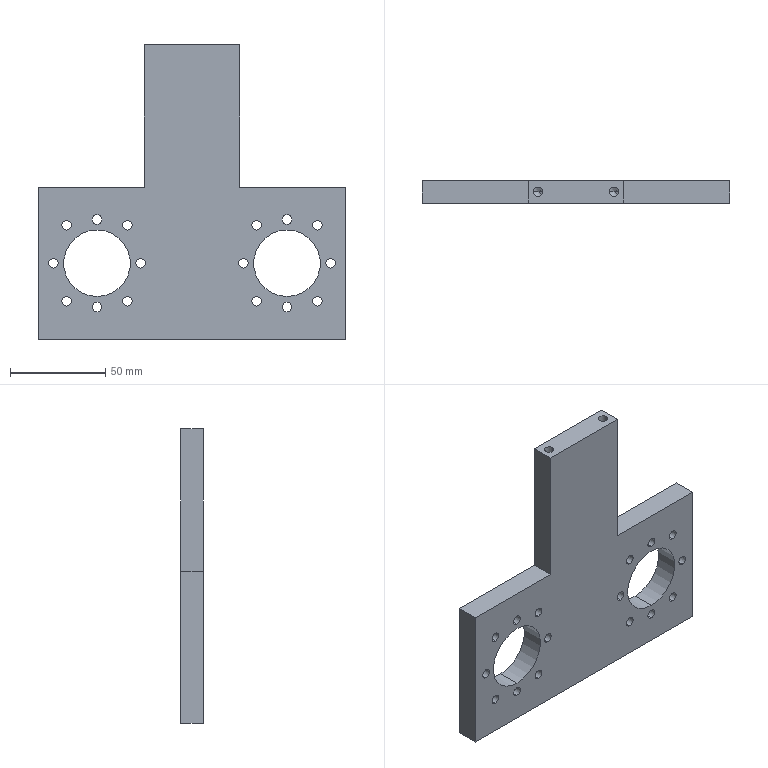Component | SolidWorks | CouplingPlate-1 | 1 solid | 54 faces | box 162 x 12 x 155 mm | volume 173051 mm3 | cylinder 40 | plane 10 | cone 4 | commonest cylinder face diameters 5 x36 35 x4
build123d program:
from build123d import *

# Parameters (mm, degrees)
SKETCH1_R                  = 17.5
EXTRUDE1_DEPTH             = 12
M6_TAPPED_HOLE1_D          = 5
M6_TAPPED_HOLE1_DEPTH      = 15
M6_TAPPED_HOLE1_TIP        = 1.502
M6_TAPPED_HOLE2_AT_2_COUNT = 2
M6_TAPPED_HOLE2_AT_2_PITCH = 32
M6_TAPPED_HOLE2_AT_3_COUNT = 2
M6_TAPPED_HOLE2_AT_3_PITCH = 51.225
M6_TAPPED_HOLE2_AT_4_COUNT = 2
M6_TAPPED_HOLE2_AT_4_PITCH = 40
M6_TAPPED_HOLE2_AT_5_COUNT = 2
M6_TAPPED_HOLE2_AT_5_PITCH = 45.88
M6_TAPPED_HOLE2_AT_6_COUNT = 2
M6_TAPPED_HOLE2_AT_6_PITCH = 43.829
M6_TAPPED_HOLE2_AT_7_COUNT = 2
M6_TAPPED_HOLE2_AT_7_PITCH = 16.279
M6_TAPPED_HOLE2_AT_8_COUNT = 2
M6_TAPPED_HOLE2_AT_8_PITCH = 21.19


with BuildPart() as part:
    # Sketch1 → Extrude1 (new body)
    with BuildSketch(Plane(origin=(0, 0, 0), x_dir=(1, 0, 0), z_dir=(0, 1, 0))):
        Polygon((-81, 80), (81, 80), (81, 0), (25, 0), (25, -75), (-25, -75), (-25, 0), (-81, 0), align=None)
        with Locations(Location((50, 40, 0), (0, 0, 270))):
            Circle(SKETCH1_R, mode=Mode.SUBTRACT)
        with Locations(Location((-50, 40, 0), (0, 0, 90))):
            Circle(SKETCH1_R, mode=Mode.SUBTRACT)
    extrude(amount=EXTRUDE1_DEPTH)

    # M6 Tapped Hole1
    with Locations(Plane.XY.offset(75)):
        with Locations((-20, 6), (20, 6)):
            Hole(M6_TAPPED_HOLE1_D / 2, depth=M6_TAPPED_HOLE1_DEPTH)
            with Locations((0, 0, -(M6_TAPPED_HOLE1_DEPTH + M6_TAPPED_HOLE1_TIP / 2))):  # 118° drill point
                Cone(0, M6_TAPPED_HOLE1_D / 2, M6_TAPPED_HOLE1_TIP, mode=Mode.SUBTRACT)

    # Sketch4 → M6 Tapped Hole2 (revolve, cut)
    with BuildSketch(Plane(origin=(-66, 12, -60), x_dir=(0, 0, 1), z_dir=(1, 0, 0))):
        Polygon((0, 0), (0, 16.502), (2.5, 15), (2.5, 0), align=None)
    m6_tapped_hole2 = revolve(axis=Axis((-66, 18.35, -60), (0, -1, 0)), mode=Mode.SUBTRACT)

    # M6 Tapped Hole2 at 2: M6 Tapped Hole2 ×2
    with Locations(*[(i * M6_TAPPED_HOLE2_AT_2_PITCH, 0, 0) for i in range(1, M6_TAPPED_HOLE2_AT_2_COUNT)]):
        add(m6_tapped_hole2, mode=Mode.SUBTRACT)

    # M6 Tapped Hole2 at 3: M6 Tapped Hole2 ×2
    with Locations(*[Vector(0.6247, 0, 0.7809) * (i * M6_TAPPED_HOLE2_AT_3_PITCH) for i in range(1, M6_TAPPED_HOLE2_AT_3_COUNT)]):
        add(m6_tapped_hole2, mode=Mode.SUBTRACT)

    # M6 Tapped Hole2 at 4: M6 Tapped Hole2 ×2
    with Locations(*[(0, 0, i * M6_TAPPED_HOLE2_AT_4_PITCH) for i in range(1, M6_TAPPED_HOLE2_AT_4_COUNT)]):
        add(m6_tapped_hole2, mode=Mode.SUBTRACT)

    # M6 Tapped Hole2 at 5: M6 Tapped Hole2 ×2
    with Locations(*[Vector(0.3487, 0, 0.9372) * (i * M6_TAPPED_HOLE2_AT_5_PITCH) for i in range(1, M6_TAPPED_HOLE2_AT_5_COUNT)]):
        add(m6_tapped_hole2, mode=Mode.SUBTRACT)

    # M6 Tapped Hole2 at 6: M6 Tapped Hole2 ×2
    with Locations(*[Vector(0.8898, 0, 0.4563) * (i * M6_TAPPED_HOLE2_AT_6_PITCH) for i in range(1, M6_TAPPED_HOLE2_AT_6_COUNT)]):
        add(m6_tapped_hole2, mode=Mode.SUBTRACT)

    # M6 Tapped Hole2 at 7: M6 Tapped Hole2 ×2
    with Locations(*[Vector(0.9829, 0, -0.1843) * (i * M6_TAPPED_HOLE2_AT_7_PITCH) for i in range(1, M6_TAPPED_HOLE2_AT_7_COUNT)]):
        add(m6_tapped_hole2, mode=Mode.SUBTRACT)

    # M6 Tapped Hole2 at 8: M6 Tapped Hole2 ×2
    with Locations(*[Vector(-0.3304, 0, 0.9439) * (i * M6_TAPPED_HOLE2_AT_8_PITCH) for i in range(1, M6_TAPPED_HOLE2_AT_8_COUNT)]):
        add(m6_tapped_hole2, mode=Mode.SUBTRACT)

    # Mirror1: M6 Tapped Hole2 across plane
    add(m6_tapped_hole2.mirror(Plane(origin=(0, 0, 0), x_dir=(0, 0, 1), z_dir=(1, 0, 0))), mode=Mode.SUBTRACT)

    # Mirror1 copy 1 sketch → Mirror1 copy 1 (revolve, cut)
    with BuildSketch(Plane(origin=(34, 12, -60), x_dir=(0, 0, 1), z_dir=(-1, 0, 0))):
        Polygon((0, 0), (0, -16.502), (2.5, -15), (2.5, 0), align=None)
    revolve(axis=Axis((34, 18.35, -60), (0, 1, 0)), mode=Mode.SUBTRACT)

    # Mirror1 copy 2 sketch → Mirror1 copy 2 (revolve, cut)
    with BuildSketch(Plane(origin=(34, 12, -20), x_dir=(0, 0, 1), z_dir=(-1, 0, 0))):
        Polygon((0, 0), (0, -16.502), (2.5, -15), (2.5, 0), align=None)
    revolve(axis=Axis((34, 18.35, -20), (0, 1, 0)), mode=Mode.SUBTRACT)

    # Mirror1 copy 3 sketch → Mirror1 copy 3 (revolve, cut)
    with BuildSketch(Plane(origin=(66, 12, -20), x_dir=(0, 0, 1), z_dir=(-1, 0, 0))):
        Polygon((0, 0), (0, -16.502), (2.5, -15), (2.5, 0), align=None)
    revolve(axis=Axis((66, 18.35, -20), (0, 1, 0)), mode=Mode.SUBTRACT)

    # Mirror1 copy 4 sketch → Mirror1 copy 4 (revolve, cut)
    with BuildSketch(Plane(origin=(50, 12, -17), x_dir=(0, 0, 1), z_dir=(-1, 0, 0))):
        Polygon((0, 0), (0, -16.502), (2.5, -15), (2.5, 0), align=None)
    revolve(axis=Axis((50, 18.35, -17), (0, 1, 0)), mode=Mode.SUBTRACT)

    # Mirror1 copy 5 sketch → Mirror1 copy 5 (revolve, cut)
    with BuildSketch(Plane(origin=(27, 12, -40), x_dir=(0, 0, 1), z_dir=(-1, 0, 0))):
        Polygon((0, 0), (0, -16.502), (2.5, -15), (2.5, 0), align=None)
    revolve(axis=Axis((27, 18.35, -40), (0, 1, 0)), mode=Mode.SUBTRACT)

    # Mirror1 copy 6 sketch → Mirror1 copy 6 (revolve, cut)
    with BuildSketch(Plane(origin=(50, 12, -63), x_dir=(0, 0, 1), z_dir=(-1, 0, 0))):
        Polygon((0, 0), (0, -16.502), (2.5, -15), (2.5, 0), align=None)
    revolve(axis=Axis((50, 18.35, -63), (0, 1, 0)), mode=Mode.SUBTRACT)

    # Mirror1 copy 7 sketch → Mirror1 copy 7 (revolve, cut)
    with BuildSketch(Plane(origin=(73, 12, -40), x_dir=(0, 0, 1), z_dir=(-1, 0, 0))):
        Polygon((0, 0), (0, -16.502), (2.5, -15), (2.5, 0), align=None)
    revolve(axis=Axis((73, 18.35, -40), (0, 1, 0)), mode=Mode.SUBTRACT)


solid = part.part

# Placed as in the assembly
solid = solid.moved(Location((-160.944, 536.983, 237.789), (0, 0, 0)))